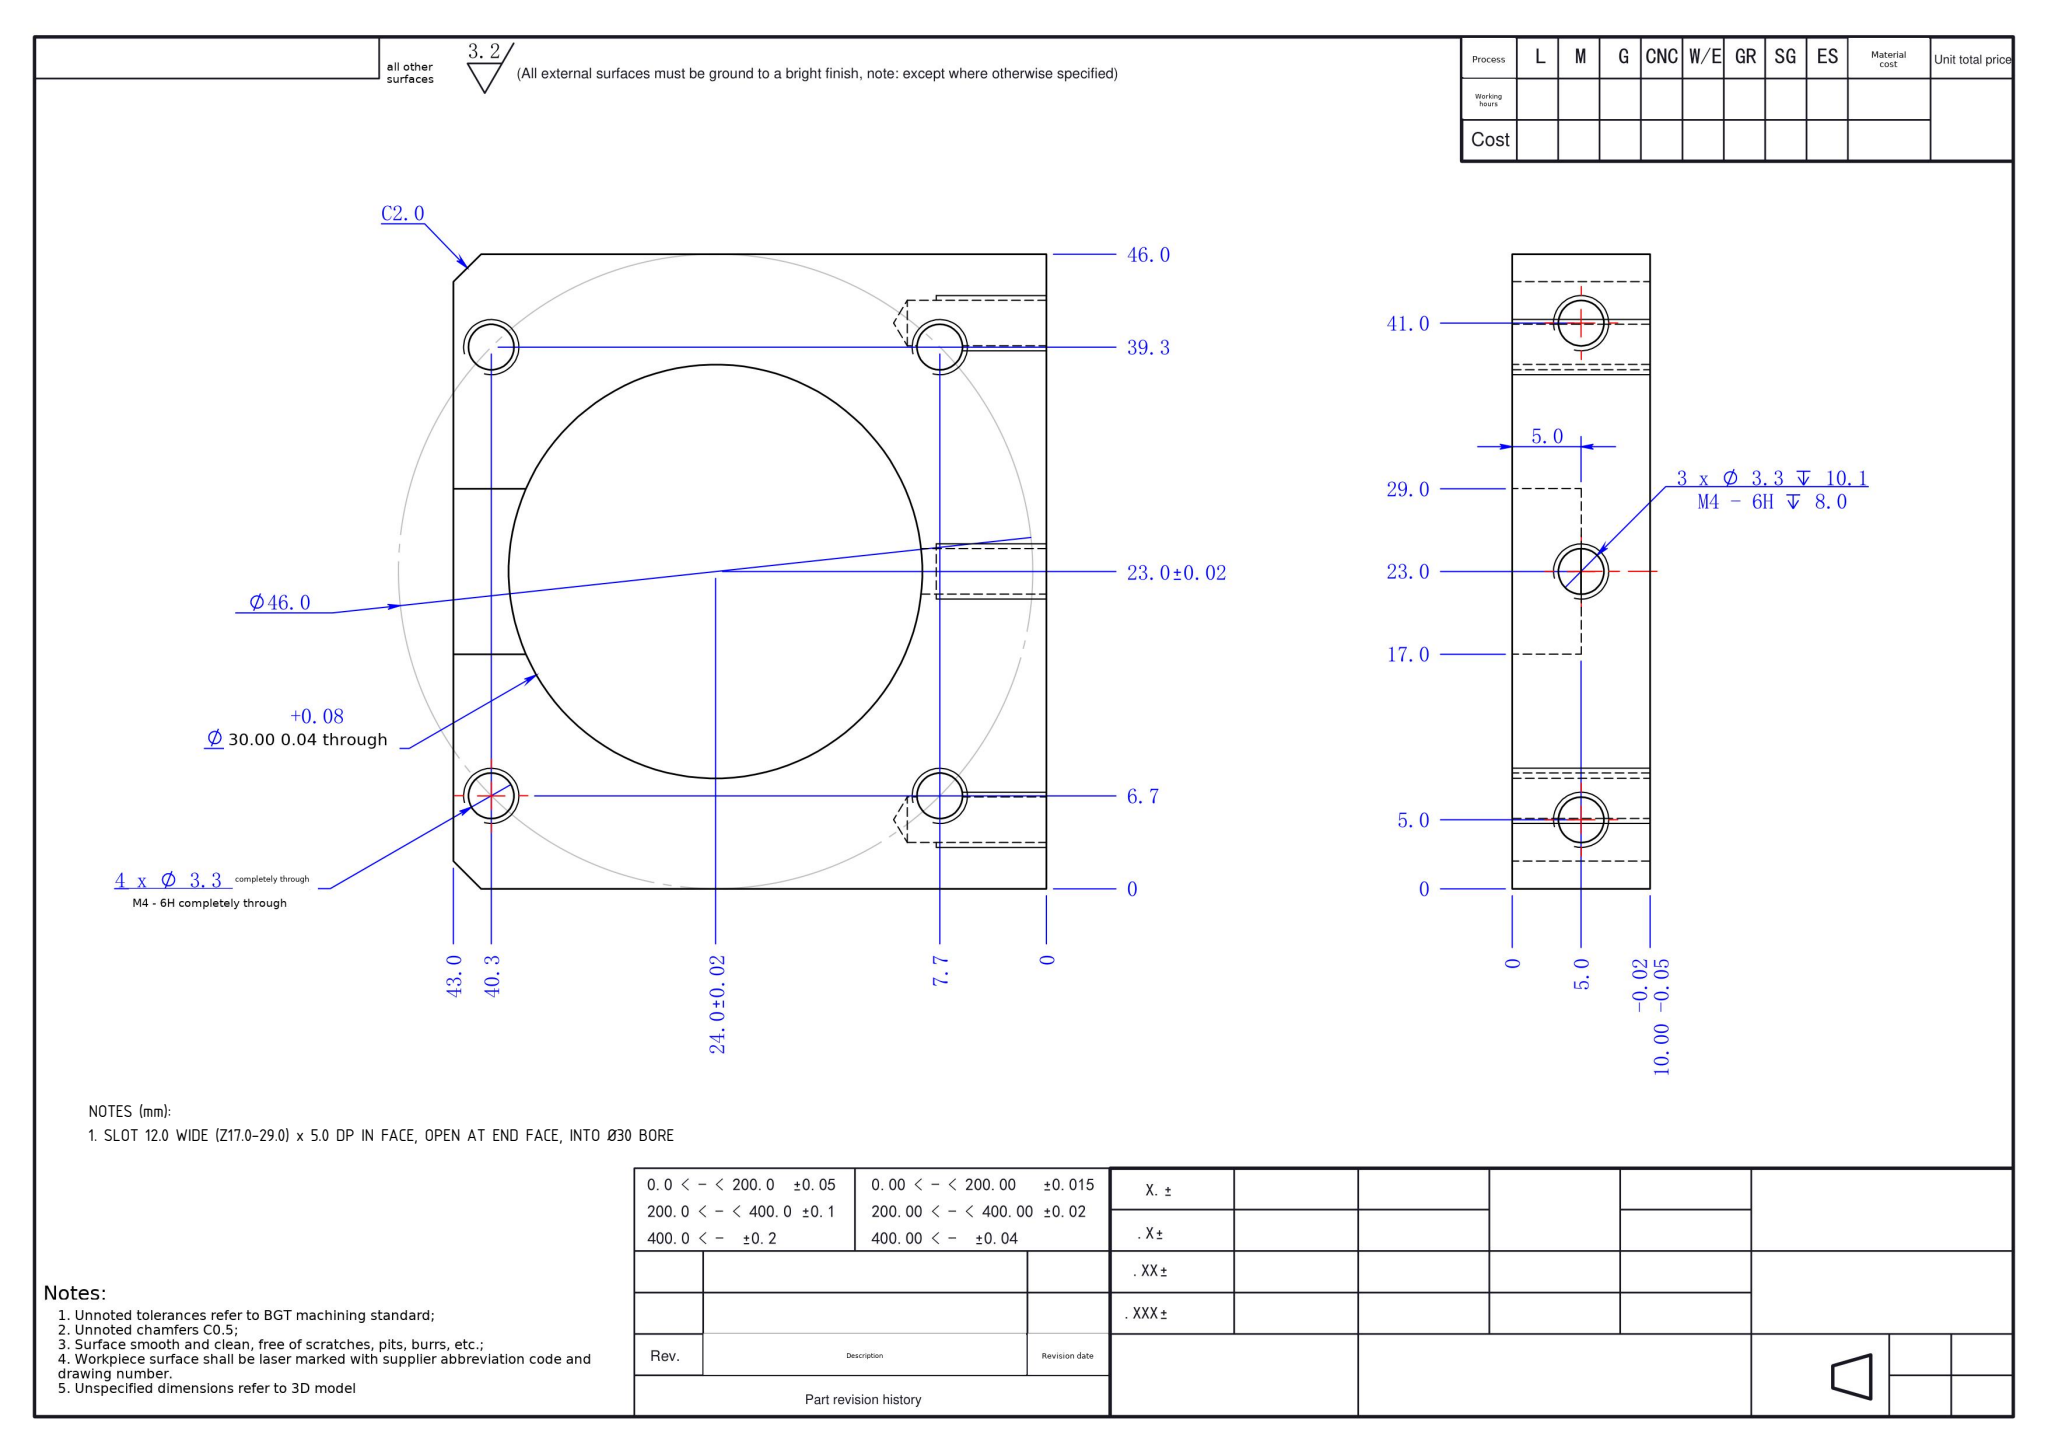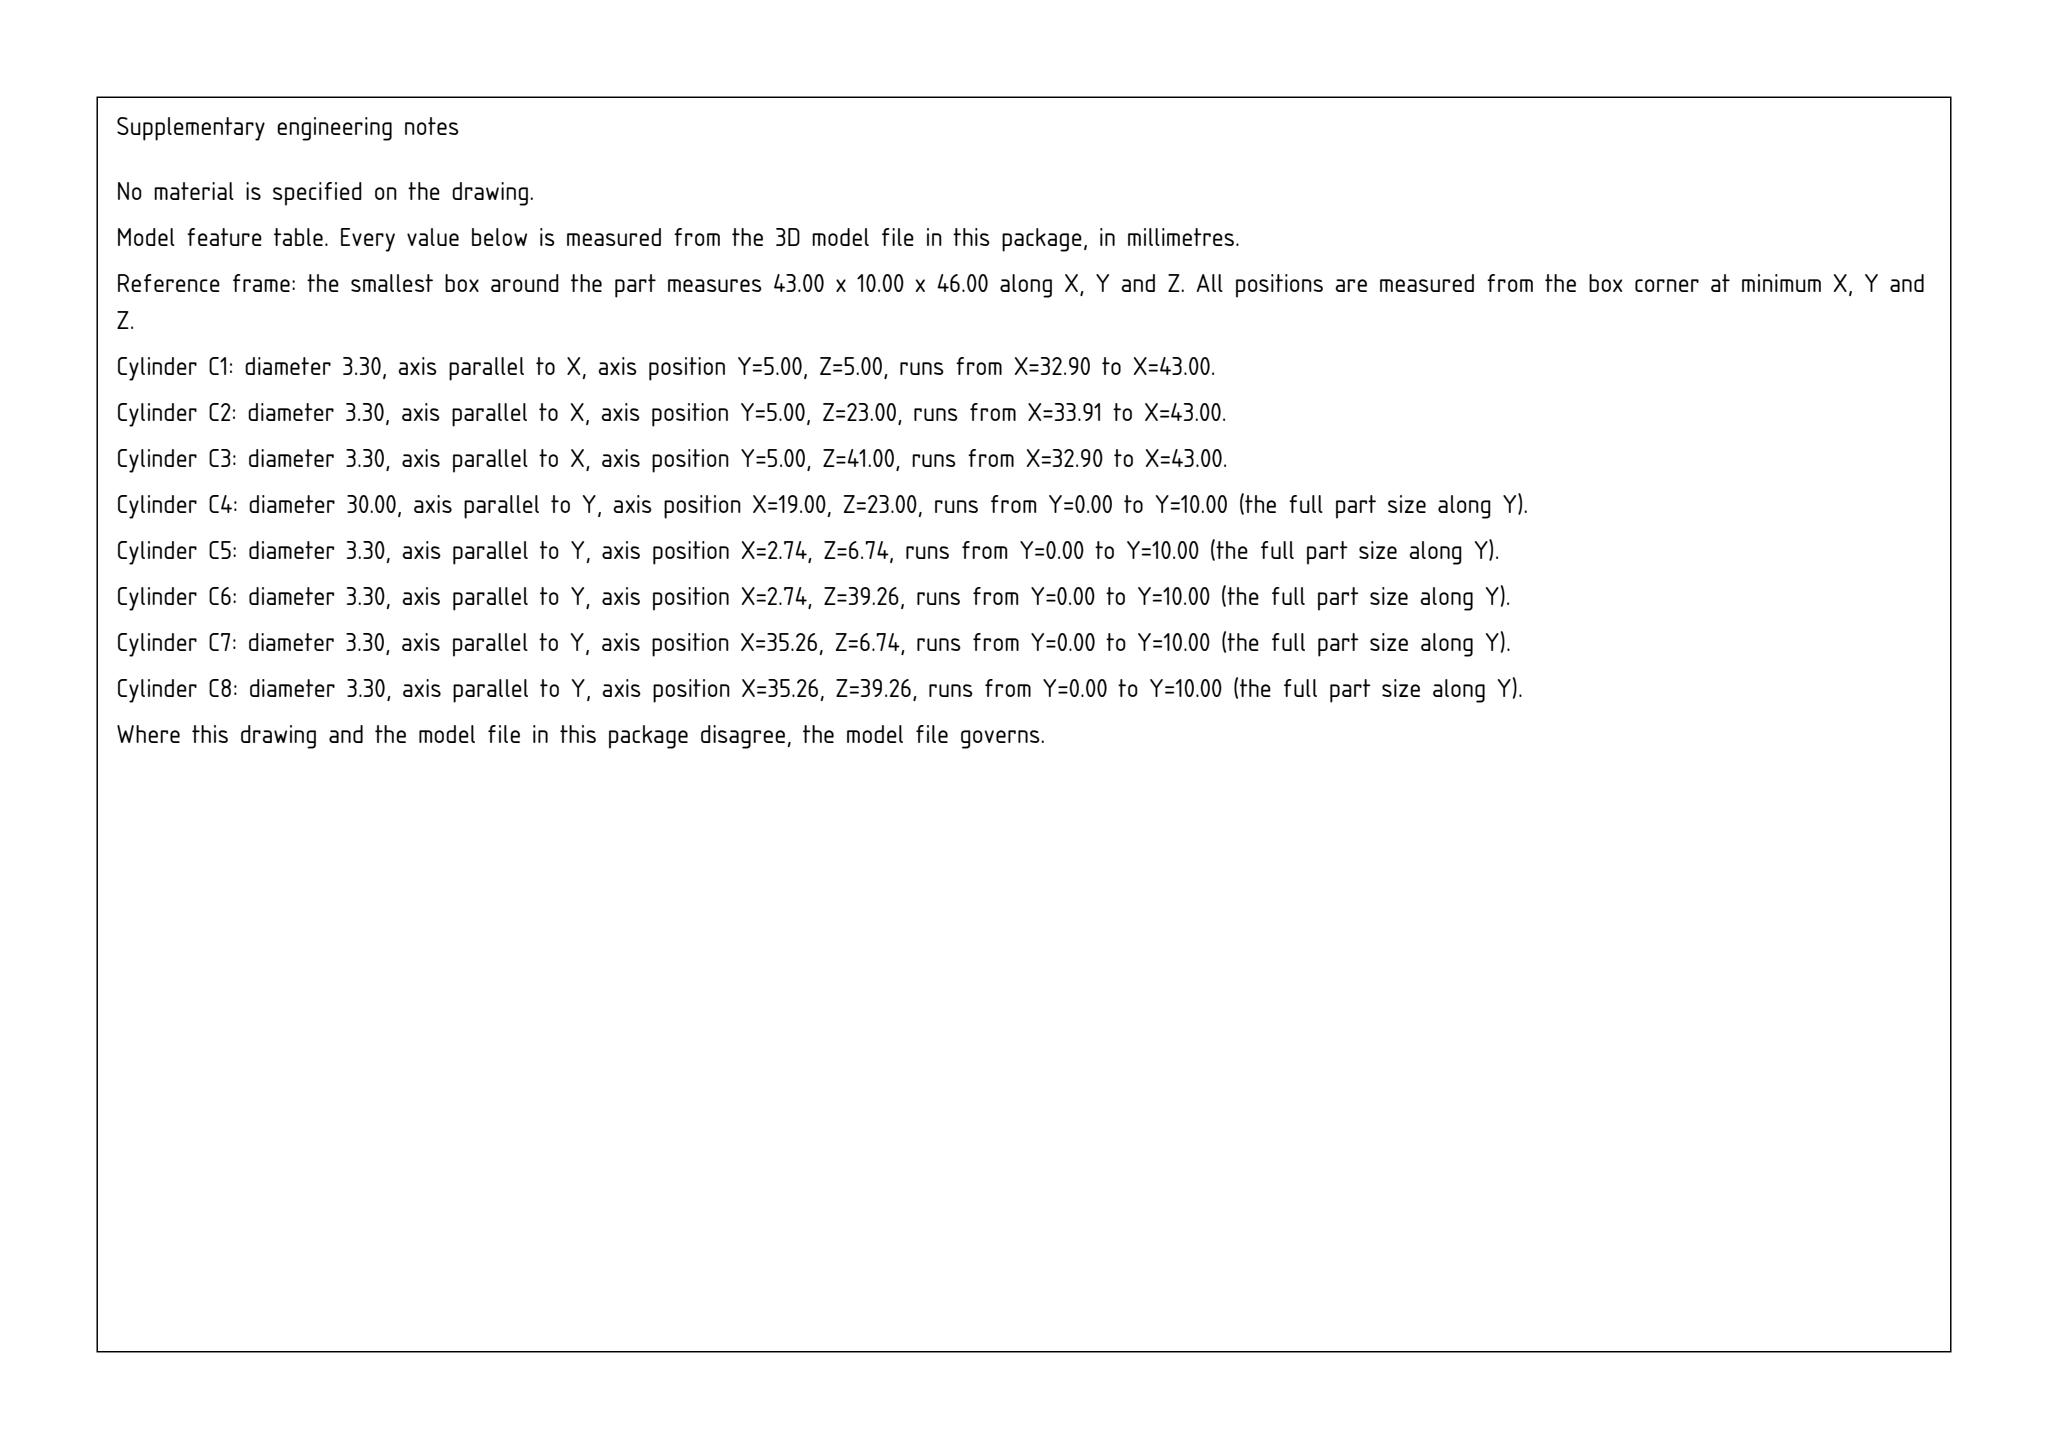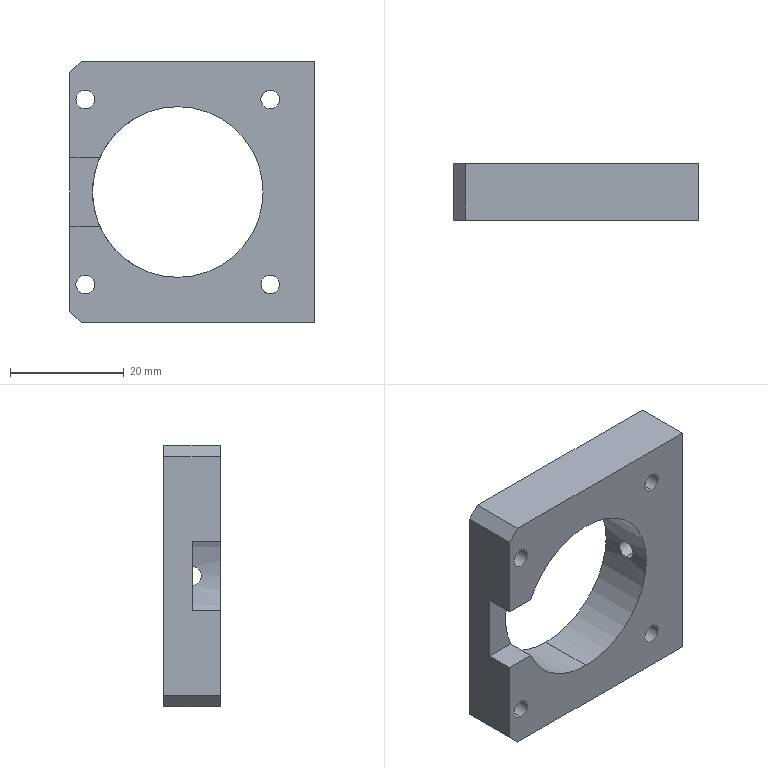Part | SolidWorks | mm | 1 solid | 31 faces | box 43 x 10 x 46 mm | volume 11828 mm3 | cylinder 16 | plane 11 | cone 4 | commonest cylinder face diameters 3.3 x14 30 x2
Drawing notes:
SLOT 12.0 WIDE (Z17.0-29.0) x 5.0 DP IN FACE, OPEN AT END FACE, INTO Ø30 BORE | from the solid: Z planes 17.0 & 29.0 (12.0 apart), Y floor plane 5.0 from Y0 face, breaks out at X end face (X0.0/43.0); no terminating X plane, runs into Ø30.0 Y-axis bore at x=19.0, z=23.0
build123d program:
from build123d import *

# Parameters (mm, degrees)
SKETCH1_W             = 43
SKETCH1_H             = 46
BOSS_EXTRUDE1_DEPTH   = 10
SKETCH2_R             = 15
CUT_EXTRUDE1_DEPTH    = 34.034
SKETCH3_W             = 10
SKETCH3_H             = 12
CUT_EXTRUDE2_DEPTH    = 5
CHAMFER1_SIZE         = 2
M4_TAPPED_HOLE1_D     = 3.3
M4_TAPPED_HOLE1_DEPTH = 10.1
M4_TAPPED_HOLE1_TIP   = 0.9914
M4_TAPPED_HOLE2_D     = 3.3
CIRPATTERN1_COUNT     = 4


with BuildPart() as part:
    # Sketch1 → Boss-Extrude1 (new body)
    with BuildSketch(Plane(origin=(0, 0, 0), x_dir=(1, 0, 0), z_dir=(0, 1, 0))):
        Rectangle(SKETCH1_W, SKETCH1_H)
    extrude(amount=BOSS_EXTRUDE1_DEPTH)

    # Sketch2 → Cut-Extrude1 (cut, through all)
    with BuildSketch(Plane(origin=(0, 10, 0), x_dir=(1, 0, 0), z_dir=(0, 1, 0))):
        with Locations(Location((-2.5, 0, 0), (0, 0, 270))):
            Circle(SKETCH2_R)
    extrude(amount=-CUT_EXTRUDE1_DEPTH, mode=Mode.SUBTRACT)

    # Sketch3 → Cut-Extrude2 (cut)
    with BuildSketch(Plane(origin=(0, 0, 0), x_dir=(1, 0, 0), z_dir=(0, 1, 0))):
        with Locations((-16.5, 0)):
            Rectangle(SKETCH3_W, SKETCH3_H)
    extrude(amount=CUT_EXTRUDE2_DEPTH, mode=Mode.SUBTRACT)

    # Chamfer1
    chamfer1_edges = [part.edges().sort_by_distance(p)[0] for p in [
        (-21.5, 5, 23),
        (-21.5, 5, -23),
    ]]
    chamfer(chamfer1_edges, length=CHAMFER1_SIZE)

    # M4 Tapped Hole1
    with Locations(Plane(origin=(21.5, 0, 0), x_dir=(0, 0, -1), z_dir=(1, 0, 0))):
        with Locations((18, 5), (0, 5), (-18, 5)):
            Hole(M4_TAPPED_HOLE1_D / 2, depth=M4_TAPPED_HOLE1_DEPTH)
            with Locations((0, 0, -(M4_TAPPED_HOLE1_DEPTH + M4_TAPPED_HOLE1_TIP / 2))):  # 118° drill point
                Cone(0, M4_TAPPED_HOLE1_D / 2, M4_TAPPED_HOLE1_TIP, mode=Mode.SUBTRACT)

    # M4 Tapped Hole2 (through all)
    with Locations(Plane(origin=(0, 10, 0), x_dir=(1, 0, 0), z_dir=(0, 1, 0))):
        with Locations((-18.763, 16.263)):
            m4_tapped_hole2 = Hole(M4_TAPPED_HOLE2_D / 2)

    # CirPattern1: M4 Tapped Hole2 ×4 about axis
    cirpattern1_axis = Axis((-2.5, 0, 0), (0, 1, 0))
    for i in range(1, CIRPATTERN1_COUNT):
        add(m4_tapped_hole2.rotate(cirpattern1_axis, i * 360 / CIRPATTERN1_COUNT), mode=Mode.SUBTRACT)


solid = part.part